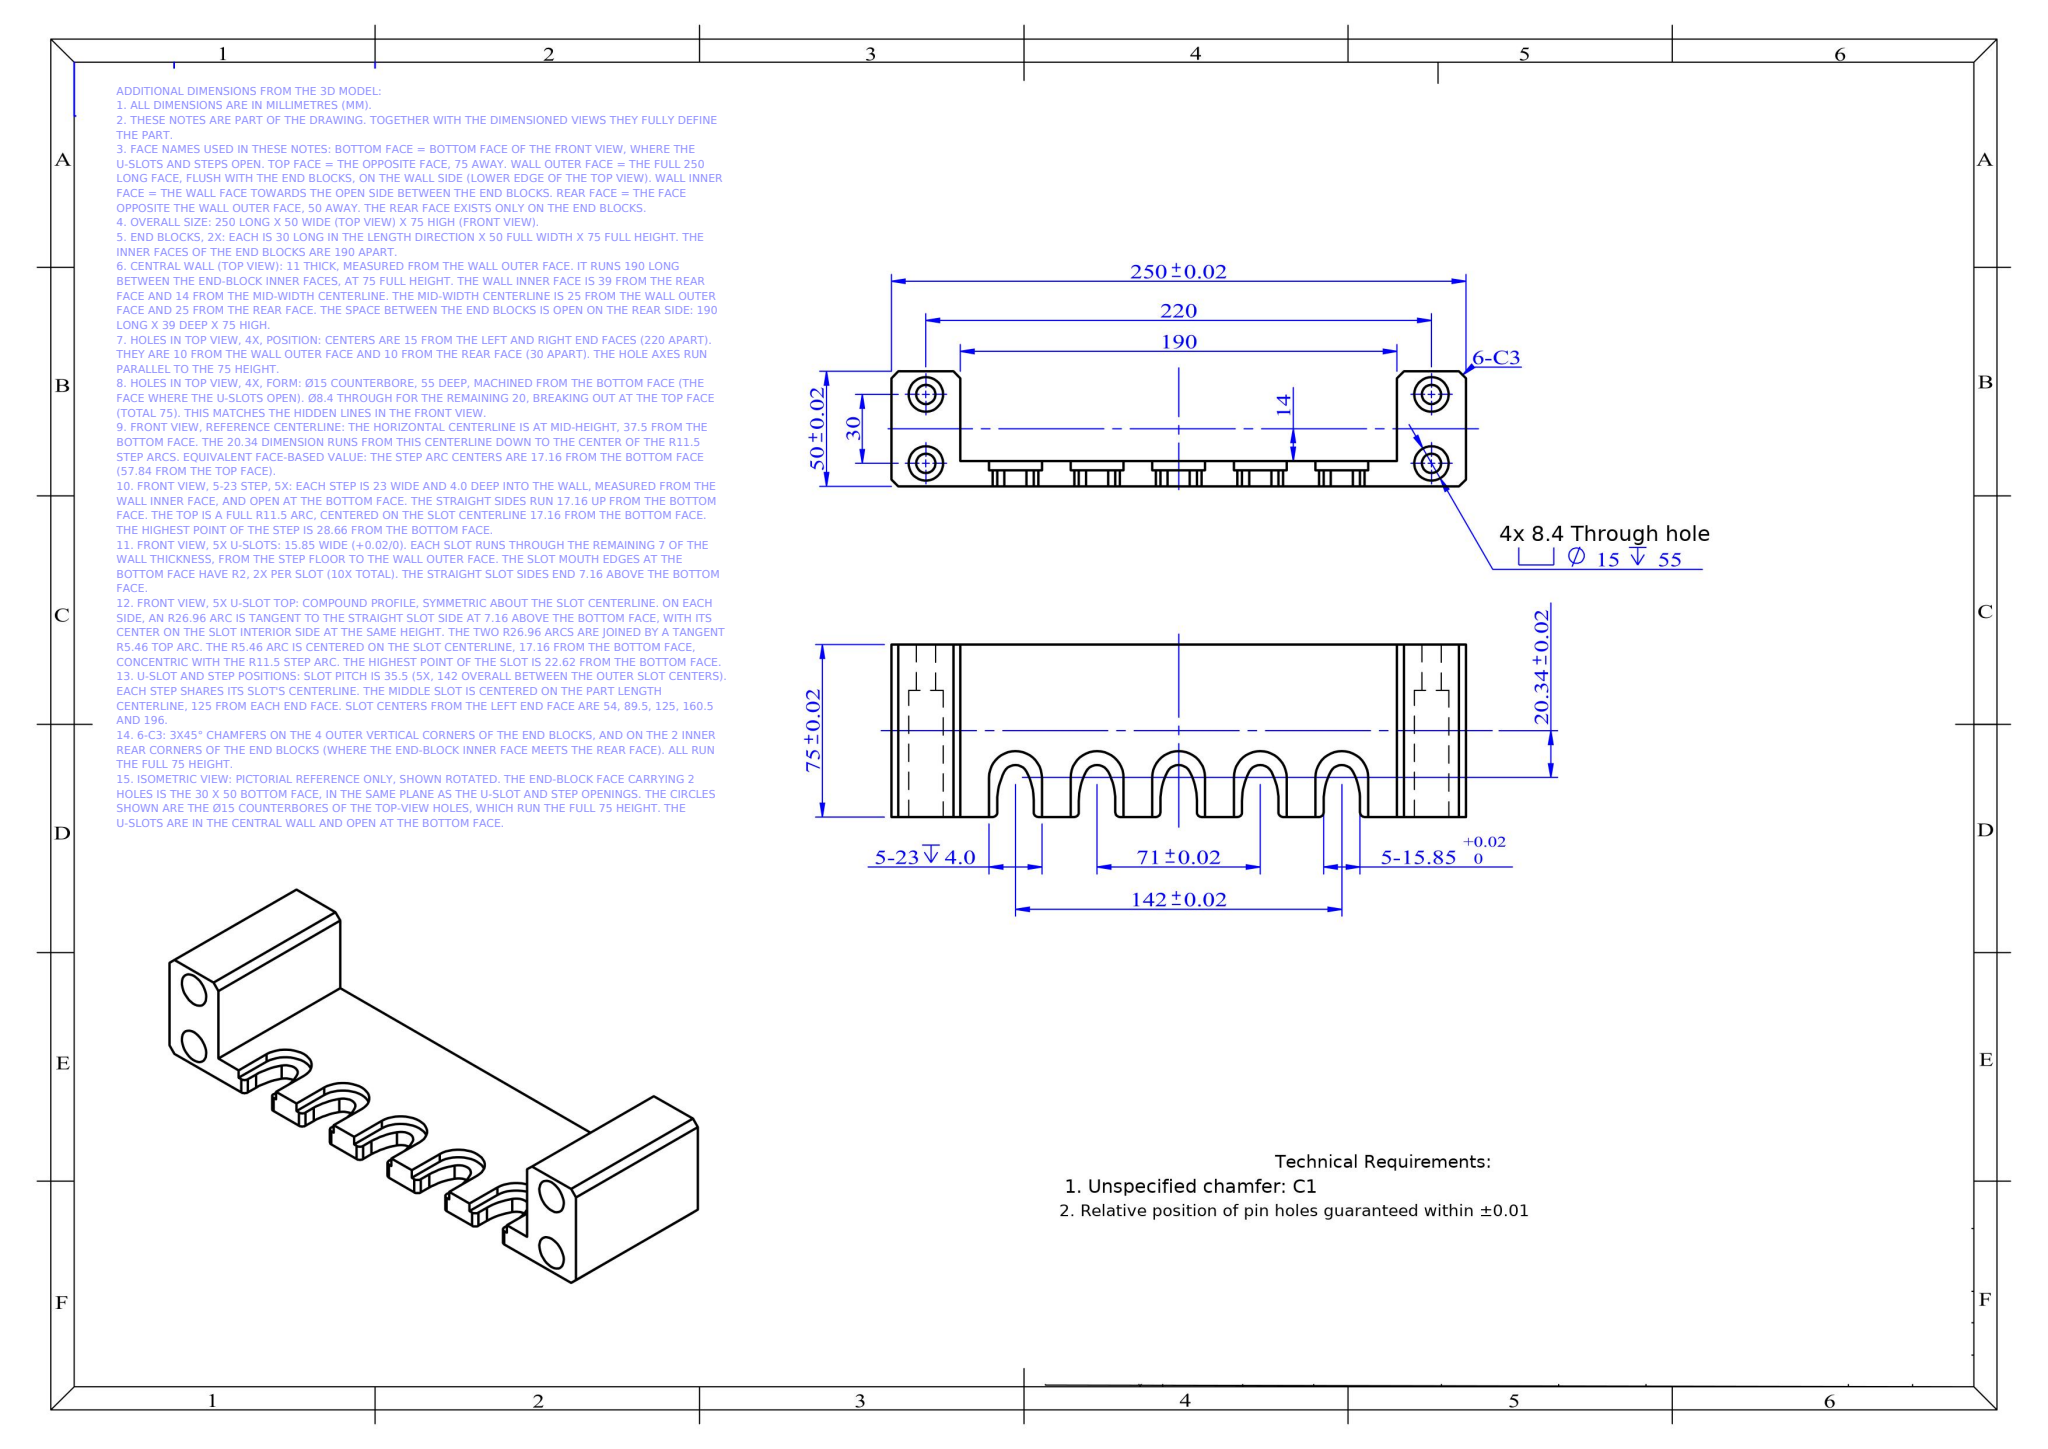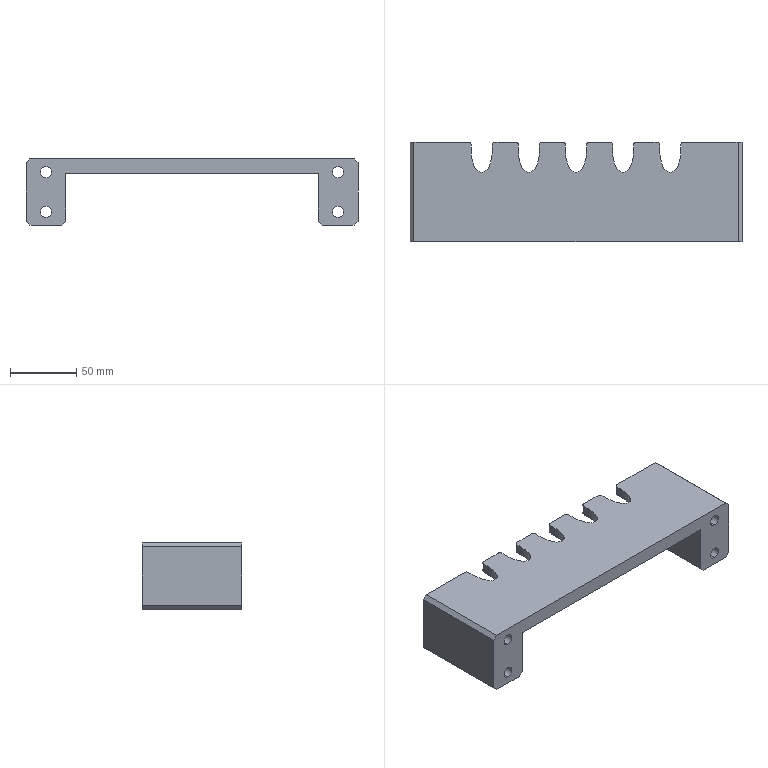Part | NX | mm | 1 solid | 96 faces | box 250 x 75 x 50 mm | volume 313555 mm3 | plane 50 | cylinder 46 | commonest cylinder face diameters 53.925 x10 4 x10 15 x8 8.4 x8 10.914 x5 23 x5